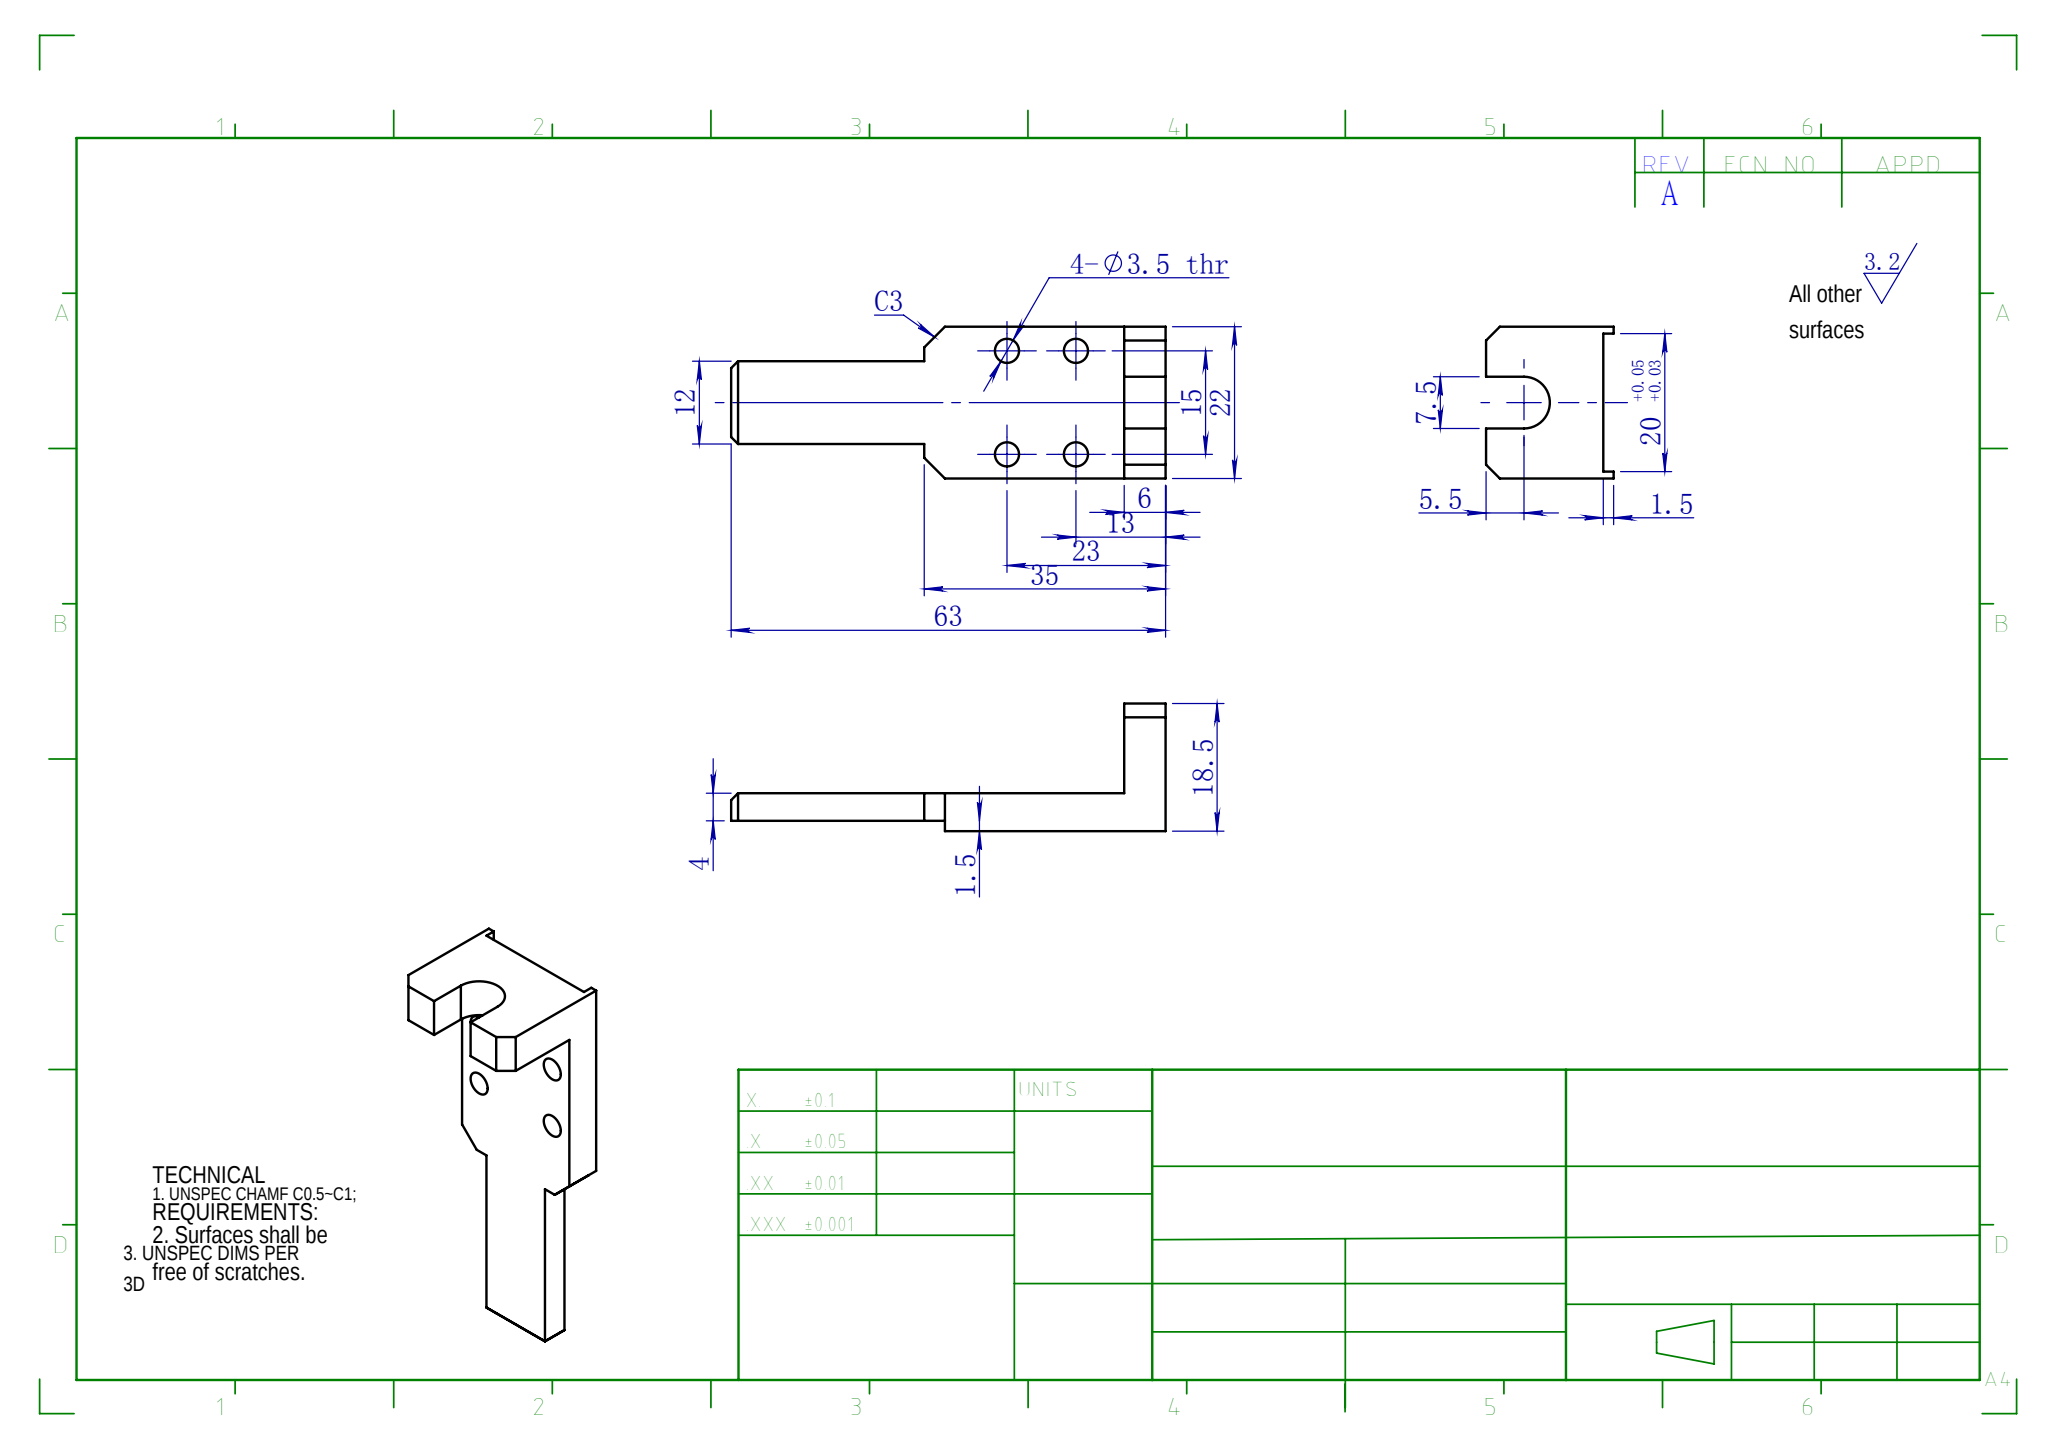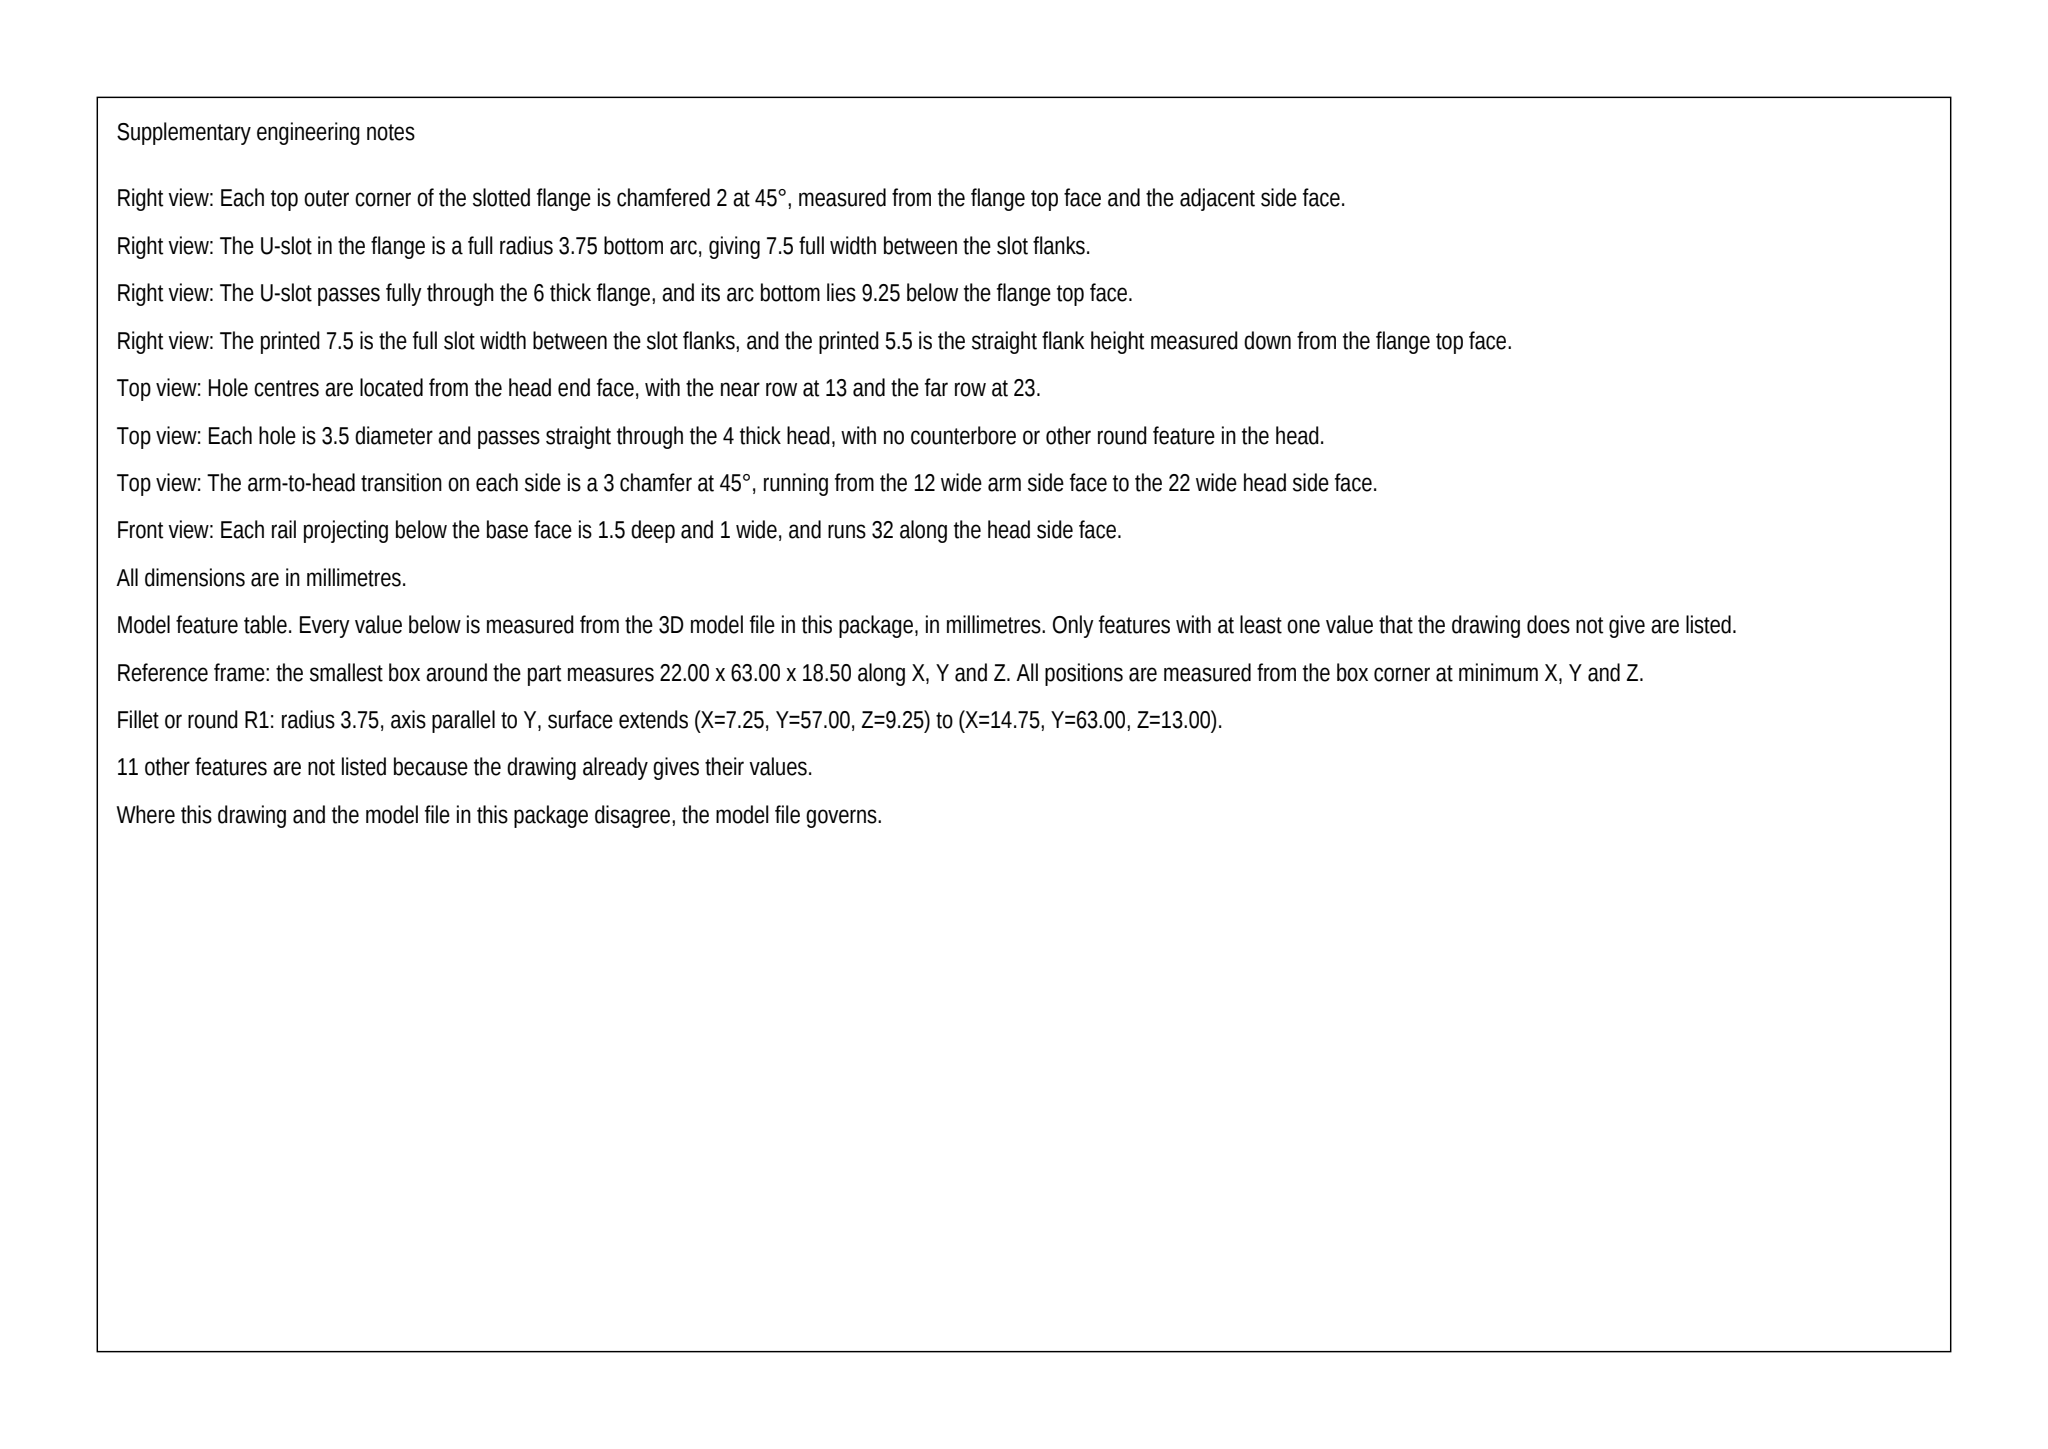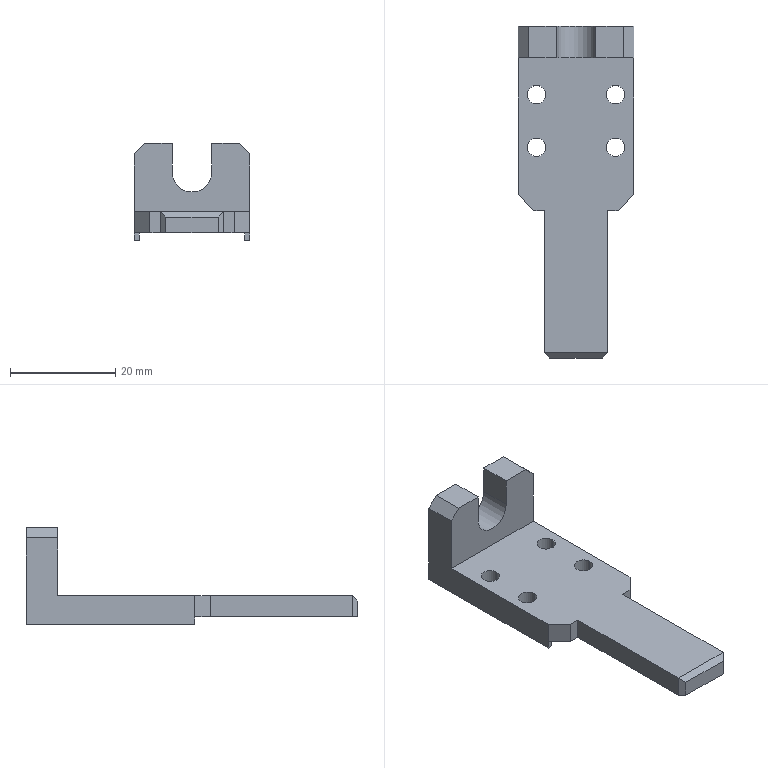Part | SolidWorks | mm | 1 solid | 37 faces | box 22 x 63 x 18.5 mm | volume 5633 mm3 | plane 28 | cylinder 9 | commonest cylinder face diameters 3.5 x8 7.5 x1
Drawing notes:
4X Ø3.5 THRU (4 THK PLATE), 15 APART, 13 & 23 FROM END | from the solid: cylinders dia 3.5 axis z, length 4.0 = full 4 plate thk; x=3.5 & 18.5 (15 apart), y=40 & 50 i.e. 23 & 13 from y=63 end
4-Ø3.5 THRU (4 THK) | from the solid: Four Ø3.5 z-axis cylinders, length 4.0, at (3.5,40),(3.5,50),(18.5,40),(18.5,50); plate z from 1.5 to 5.5 = 4 thk
build123d program:
from build123d import *

# Parameters (mm, degrees)
SKETCH1_W             = 12
SKETCH1_H             = 63
BOSS_EXTRUDE1_DEPTH   = 4
SKETCH1_2_W           = 22
SKETCH1_2_H           = 35
BOSS_EXTRUDE1_2_DEPTH = 4
SKETCH2_W             = 22
SKETCH2_H             = 6
BOSS_EXTRUDE2_DEPTH   = 13
CUT_EXTRUDE1_DEPTH    = 67.174
CHAMFER1_SIZE         = 3
CHAMFER2_SIZE         = 1
SKETCH4_R             = 1.75
CUT_EXTRUDE2_DEPTH    = 36.809
SKETCH5_W             = 1
SKETCH5_H             = 32
BOSS_EXTRUDE3_DEPTH   = 1.5
CHAMFER3_SIZE         = 2


with BuildPart() as part:
    # Sketch1 → Boss-Extrude1 (new body)
    with BuildSketch(Plane.XY):
        Rectangle(SKETCH1_W, SKETCH1_H)
    extrude(amount=BOSS_EXTRUDE1_DEPTH)

    # Sketch1_2 → Boss-Extrude1_2 (add)
    with BuildSketch(Plane(origin=(0, 0, 0), x_dir=(-1, 0, 0), z_dir=(0, 0, -1))):
        with Locations((0, 14)):
            Rectangle(SKETCH1_2_W, SKETCH1_2_H)
    extrude(amount=-BOSS_EXTRUDE1_2_DEPTH)

    # Sketch2 → Boss-Extrude2 (add)
    with BuildSketch(Plane.XY.offset(4)):
        with Locations((0, 28.5)):
            Rectangle(SKETCH2_W, SKETCH2_H)
    extrude(amount=BOSS_EXTRUDE2_DEPTH)

    # Sketch3 → Cut-Extrude1 (cut, through all)
    with BuildSketch(Plane(origin=(0, 31.5, 0), x_dir=(1, 0, 0), z_dir=(0, 1, 0))):
        with BuildLine():
            Line((-3.75, -17), (-3.75, -11.5))
            ThreePointArc((-3.75, -11.5), (0, -7.75), (3.75, -11.5))
            Line((3.75, -11.5), (3.75, -17))
            ThreePointArc((3.75, -17), (0, -20.75), (-3.75, -17))
        make_face()
    extrude(amount=-CUT_EXTRUDE1_DEPTH, mode=Mode.SUBTRACT)

    # Chamfer1
    chamfer1_edges = [part.edges().sort_by_distance(p)[0] for p in [
        (11, -3.5, 2),
        (-11, -3.5, 2),
    ]]
    chamfer(chamfer1_edges, length=CHAMFER1_SIZE)

    # Chamfer2
    chamfer2_edges = [part.edges().sort_by_distance(p)[0] for p in [
        (0, -31.5, 4),
        (6, -31.5, 2),
        (-6, -31.5, 2),
    ]]
    chamfer(chamfer2_edges, length=CHAMFER2_SIZE)

    # Sketch4 → Cut-Extrude2 (cut, through all)
    with BuildSketch(Plane.XY.offset(4)):
        with Locations((7.5, 8.5)):
            Circle(SKETCH4_R)
        with Locations((7.5, 18.5)):
            Circle(SKETCH4_R)
        with Locations((-7.5, 18.5)):
            Circle(SKETCH4_R)
        with Locations((-7.5, 8.5)):
            Circle(SKETCH4_R)
    extrude(amount=-CUT_EXTRUDE2_DEPTH, mode=Mode.SUBTRACT)

    # Sketch5 → Boss-Extrude3 (add)
    with BuildSketch(Plane(origin=(0, 0, 0), x_dir=(-1, 0, 0), z_dir=(0, 0, -1))):
        with Locations((10.5, 15.5)):
            Rectangle(SKETCH5_W, SKETCH5_H)
        with Locations((-10.5, 15.5)):
            Rectangle(SKETCH5_W, SKETCH5_H)
    extrude(amount=BOSS_EXTRUDE3_DEPTH)

    # Chamfer3
    chamfer3_edges = [part.edges().sort_by_distance(p)[0] for p in [
        (-11, 28.5, 17),
        (11, 28.5, 17),
    ]]
    chamfer(chamfer3_edges, length=CHAMFER3_SIZE)


solid = part.part